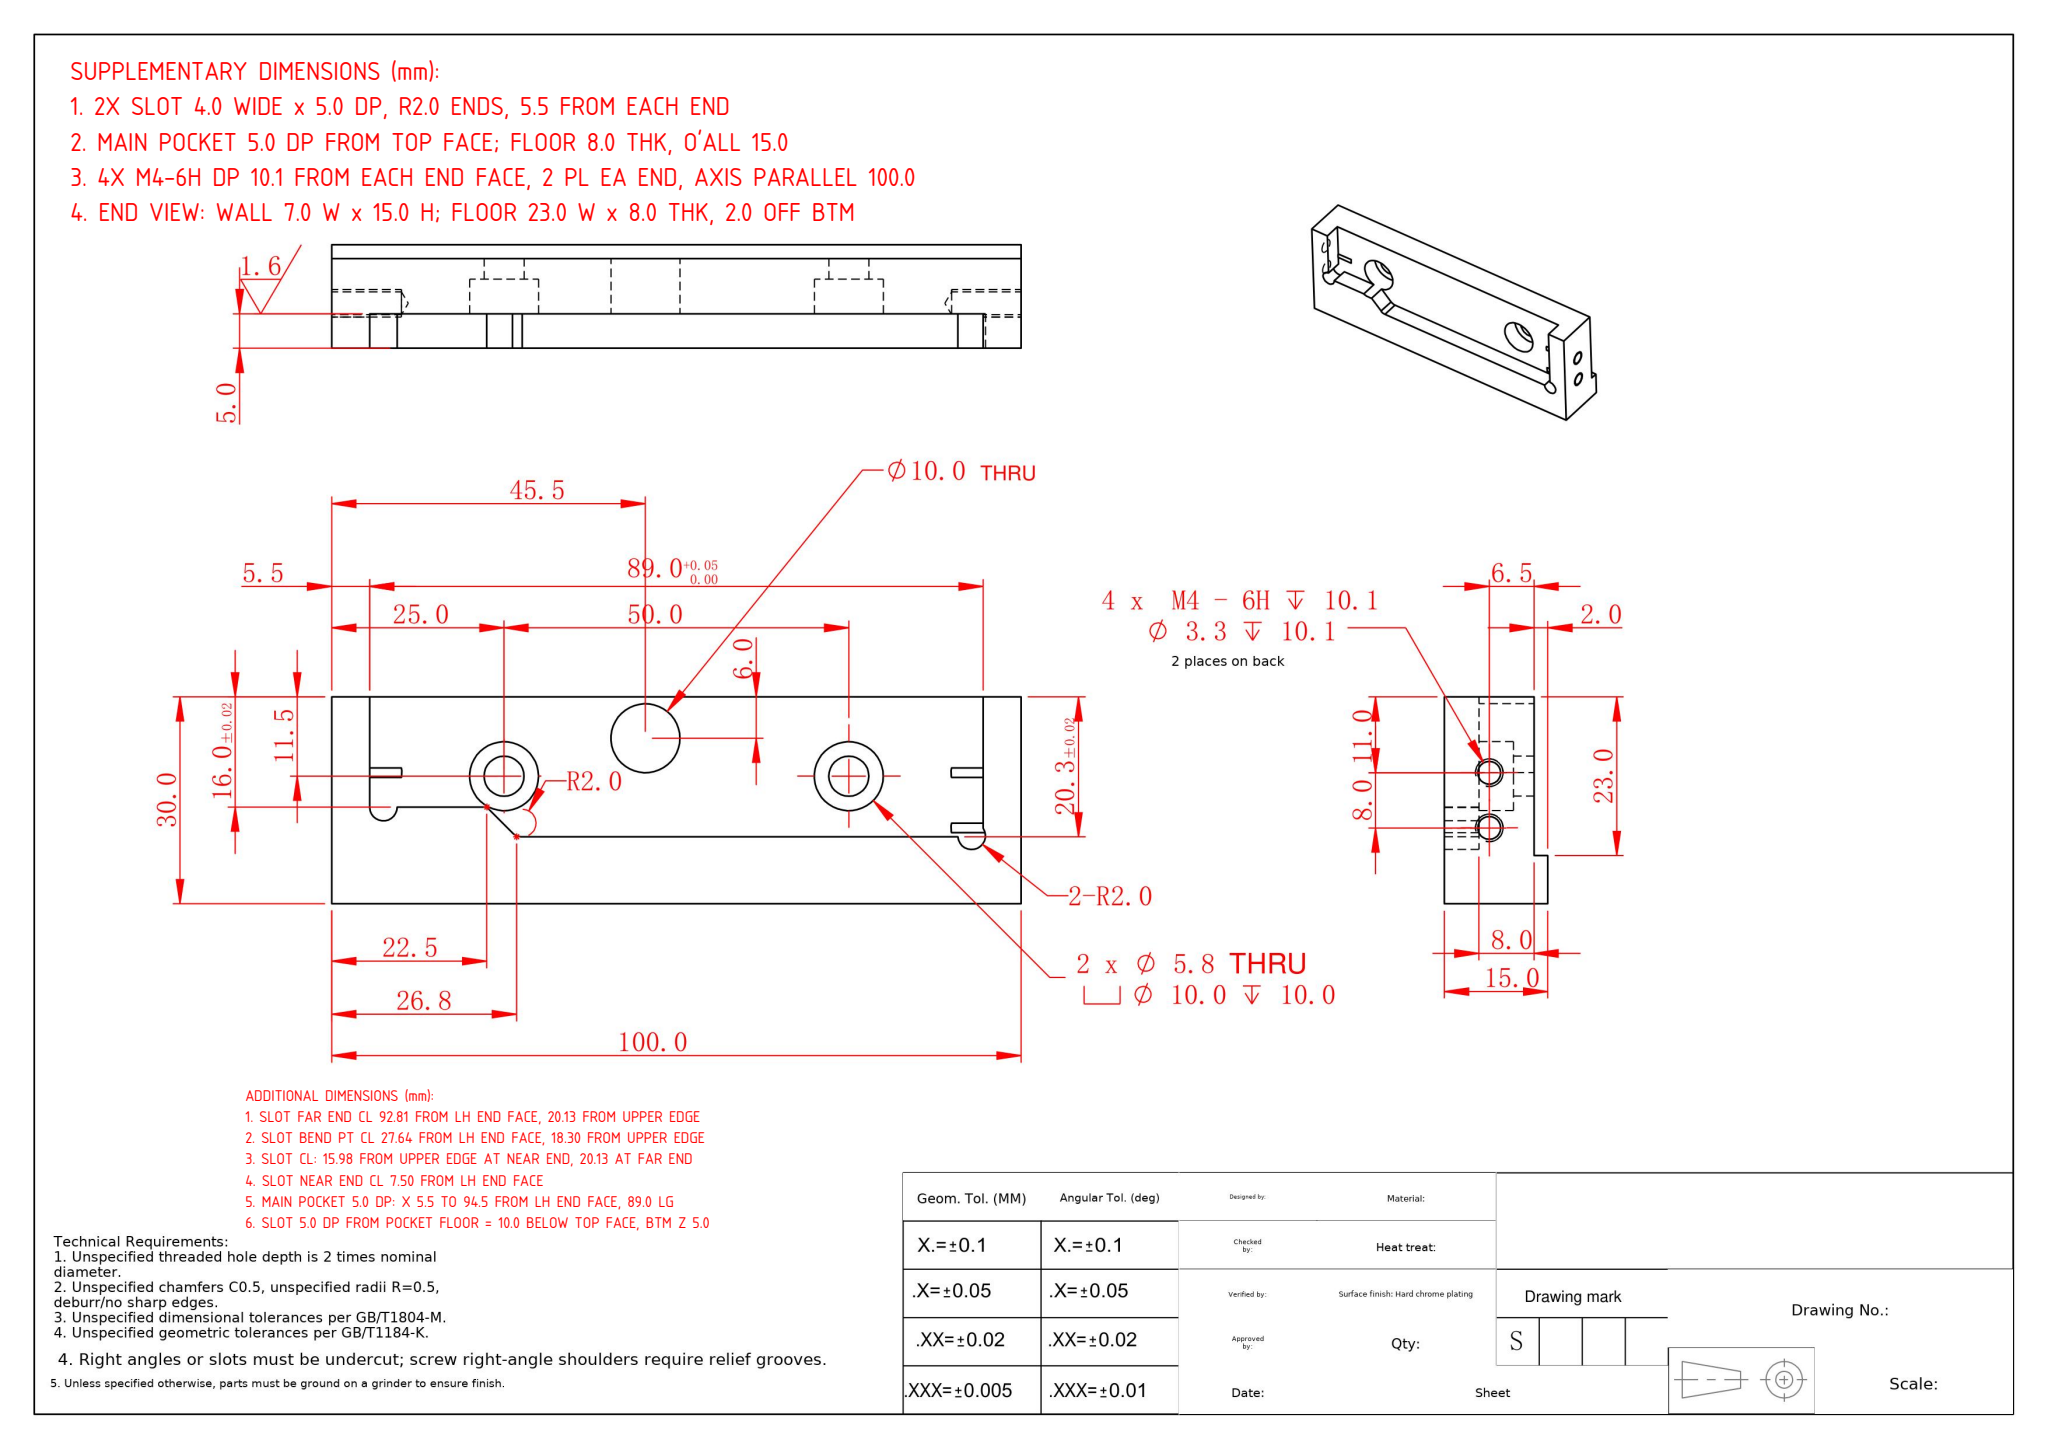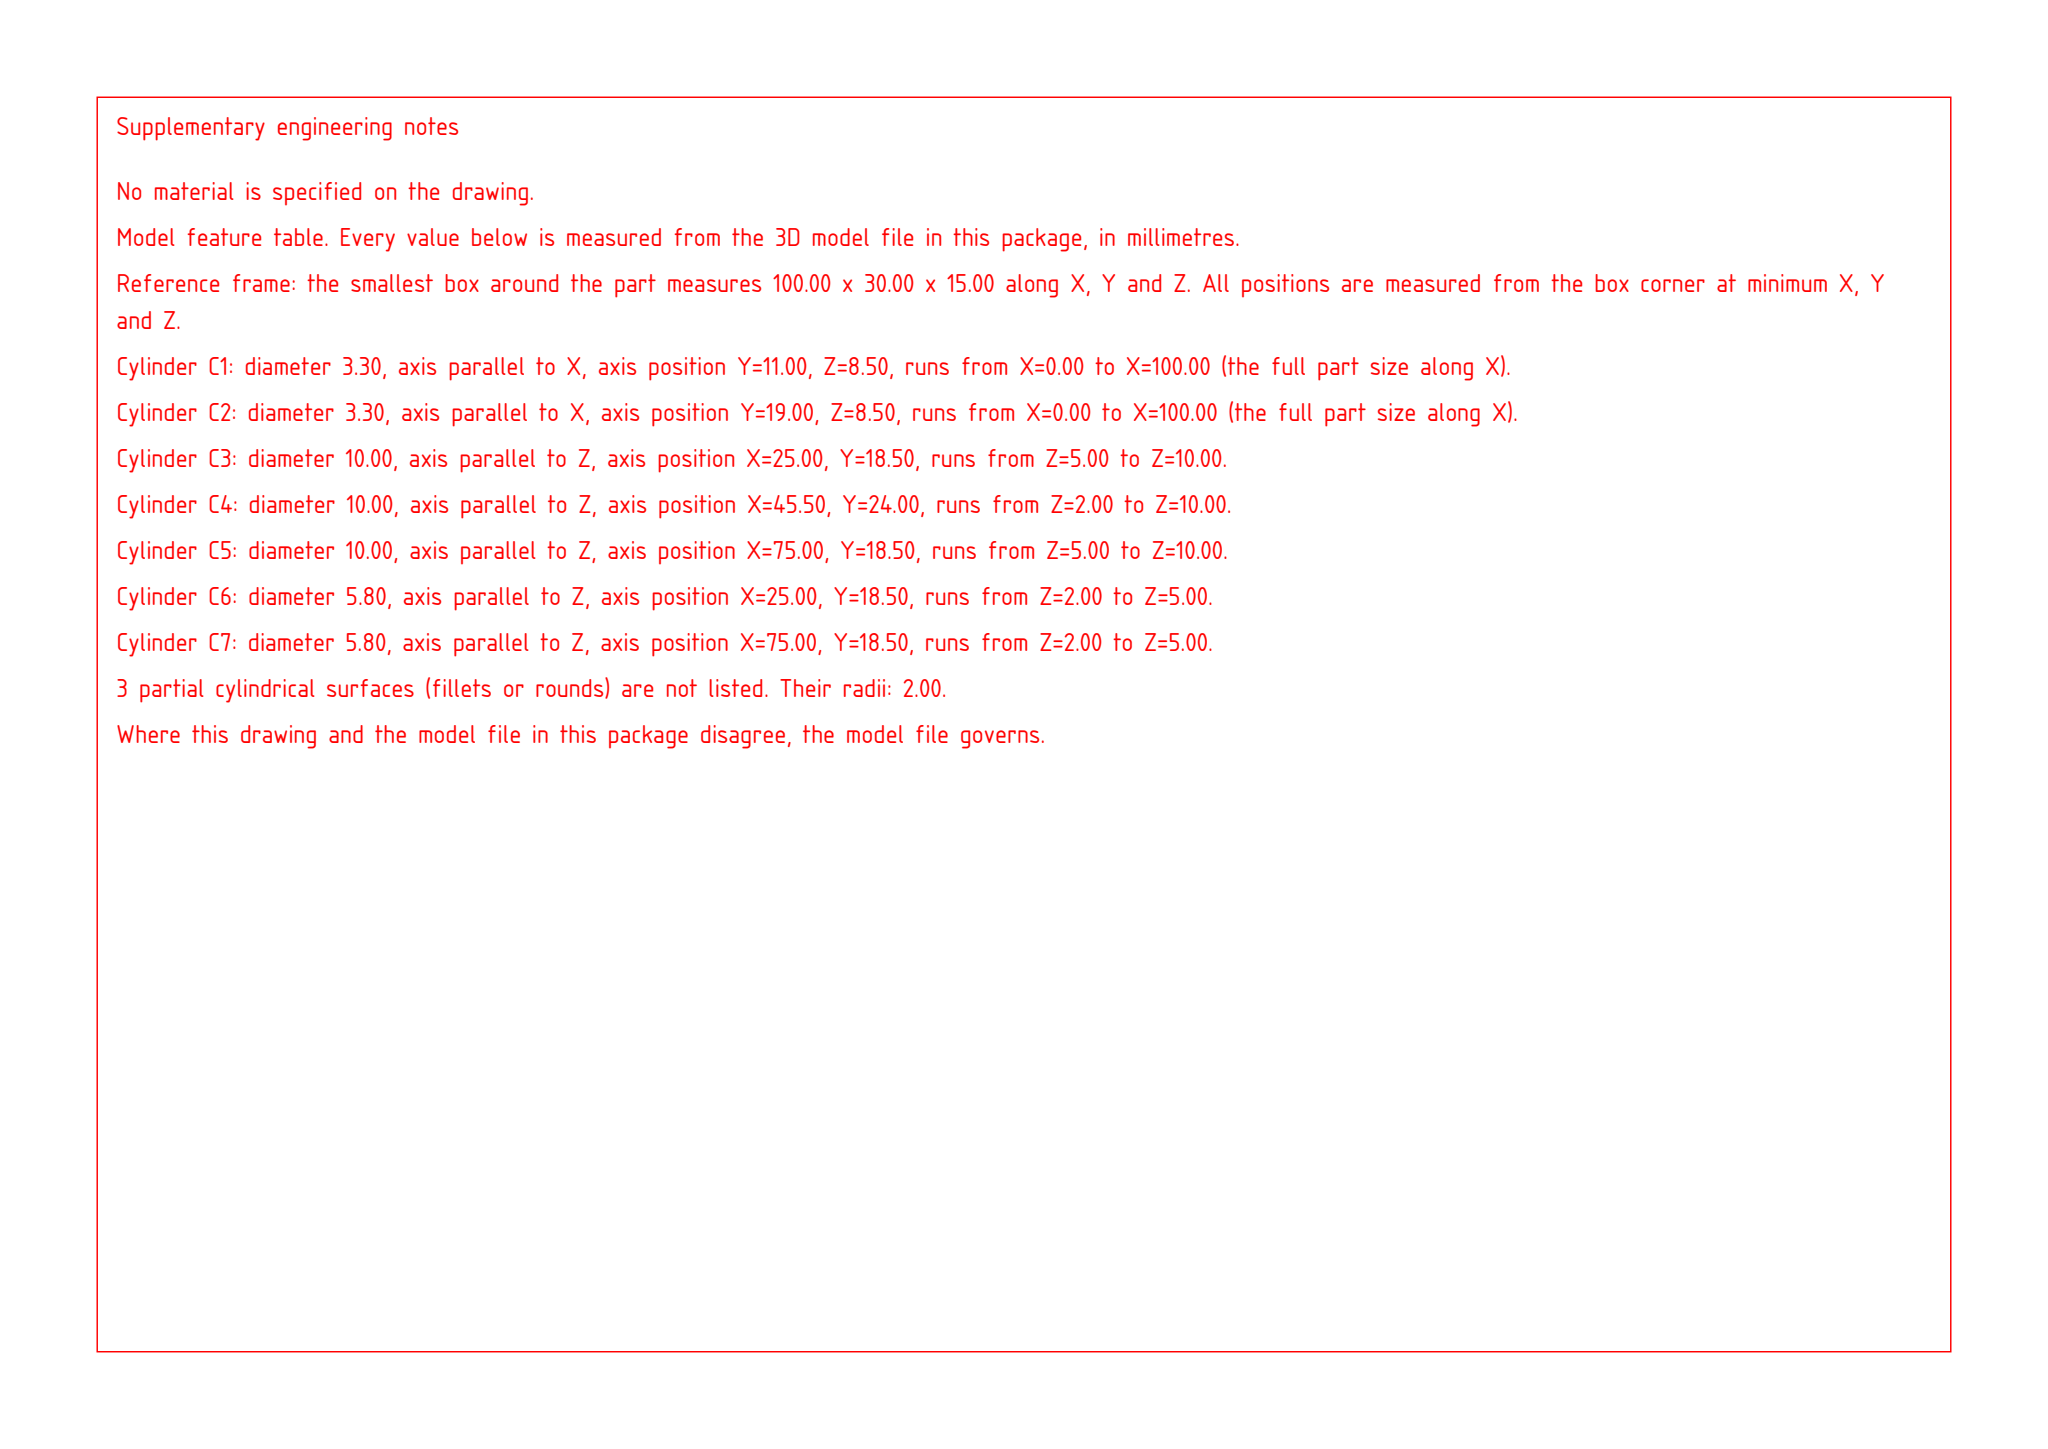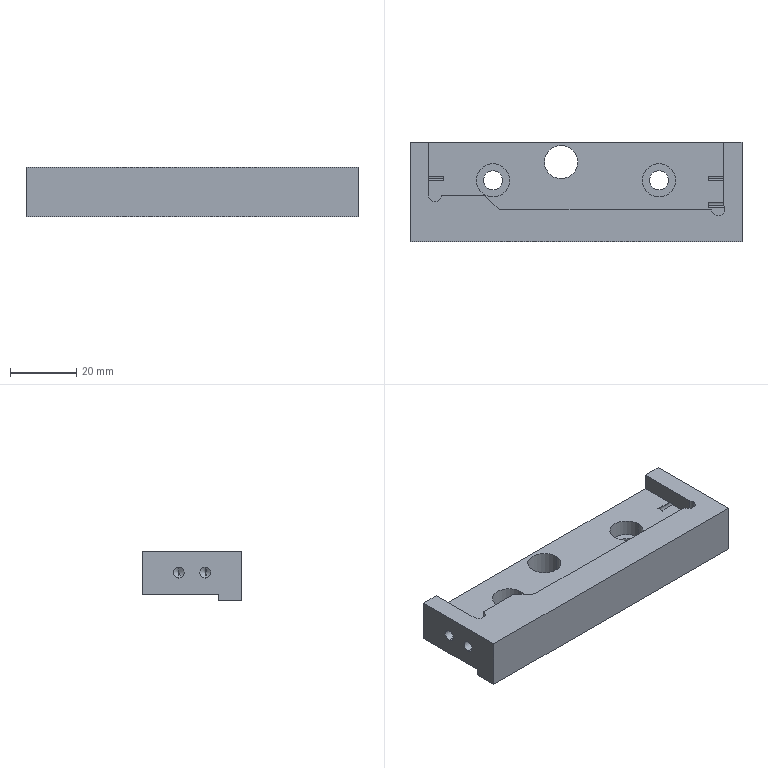Part | SolidWorks | mm | 1 solid | 46 faces | box 100 x 30 x 15 mm | volume 29792 mm3 | cylinder 22 | plane 16 | cone 8 | commonest cylinder face diameters 3.3 x8 10 x6 5.8 x4 4 x4